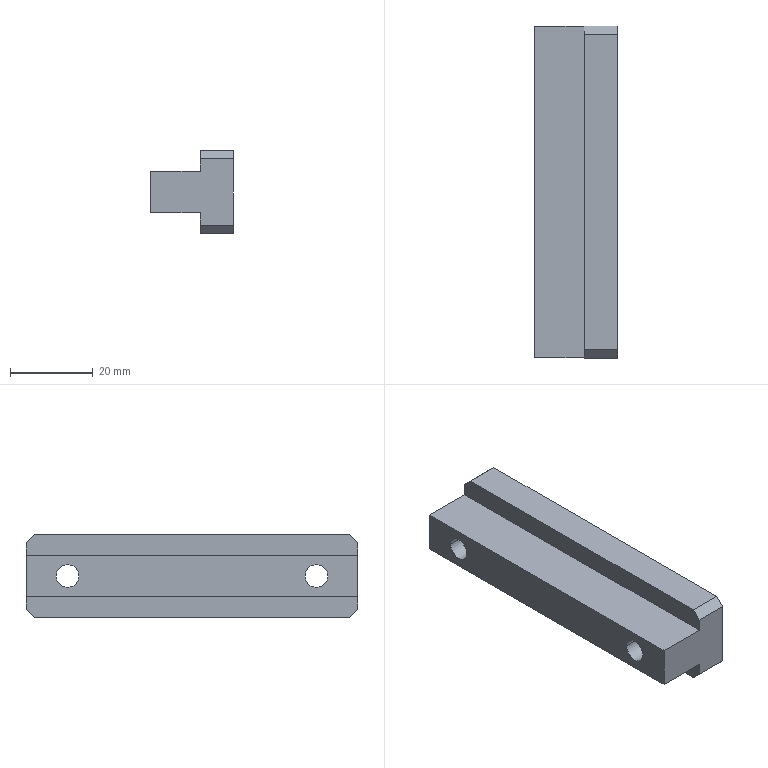Component | SolidWorks | ClampingAssembly-1_A85-1 | 1 solid | 24 faces | box 20 x 80 x 20 mm | volume 20761 mm3 | plane 16 | cylinder 8 | commonest cylinder face diameters 10 x4 5.5 x4 | material S136
build123d program:
from build123d import *

# Parameters (mm, degrees)
SKETCH1_W                                           = 80
SKETCH1_H                                           = 15
BOSS_EXTRUDE1_DEPTH                                 = 10
SKETCH2_W                                           = 12
SKETCH2_H                                           = 5
CUT_EXTRUDE1_DEPTH                                  = 81.971
SKETCH5_W                                           = 8
SKETCH5_H                                           = 5
BOSS_EXTRUDE2_DEPTH                                 = 80
HOLE_SIZE_ACCORDING_TO_HEXAGON_SOCKET_H_D           = 5.5
HOLE_SIZE_ACCORDING_TO_HEXAGON_SOCKET_H_CBORE_D     = 10
HOLE_SIZE_ACCORDING_TO_HEXAGON_SOCKET_H_CBORE_DEPTH = 5.7
CHAMFER1_SIZE                                       = 2


with BuildPart() as part:
    # Sketch1 → Boss-Extrude1 (new, symmetric)
    with BuildSketch(Plane(origin=(0, 0, 0), x_dir=(0, 0, -1), z_dir=(1, 0, 0))):
        Rectangle(SKETCH1_W, SKETCH1_H)
    extrude(amount=BOSS_EXTRUDE1_DEPTH, both=True)

    # Sketch2 → Cut-Extrude1 (cut, through all)
    with BuildSketch(Plane(origin=(0, 0, -40), x_dir=(-1, 0, 0), z_dir=(0, 0, -1))):
        with Locations((4, -5)):
            Rectangle(SKETCH2_W, SKETCH2_H)
    extrude(amount=-CUT_EXTRUDE1_DEPTH, mode=Mode.SUBTRACT)

    # Sketch5 → Boss-Extrude2 (add)
    with BuildSketch(Plane.XY.offset(40)):
        with Locations((6, 10)):
            Rectangle(SKETCH5_W, SKETCH5_H)
    extrude(amount=-BOSS_EXTRUDE2_DEPTH)

    # Hole Size_ according to_Hexagon Socket H (through all)
    with Locations(Plane(origin=(10, 0, 0), x_dir=(0, 0, -1), z_dir=(1, 0, 0))):
        with Locations((-30, 2.5), (30, 2.5)):
            CounterBoreHole(HOLE_SIZE_ACCORDING_TO_HEXAGON_SOCKET_H_D / 2, HOLE_SIZE_ACCORDING_TO_HEXAGON_SOCKET_H_CBORE_D / 2, HOLE_SIZE_ACCORDING_TO_HEXAGON_SOCKET_H_CBORE_DEPTH)

    # Chamfer1
    chamfer1_edges = [part.edges().sort_by_distance(p)[0] for p in [
        (6, 12.5, 40),
        (6, 12.5, -40),
        (6, -7.5, -40),
        (6, -7.5, 40),
    ]]
    chamfer(chamfer1_edges, length=CHAMFER1_SIZE)


solid = part.part

# Placed as in the assembly
solid = solid.moved(Location((-4.551, 48.036, -3), (90, 0, 0)))
STEP:
#1=CARTESIAN_POINT('',(-0.009873,0.5132,-0.01969));
#2=VERTEX_POINT('',#1);
#3=CARTESIAN_POINT('',(-0.009873,0.9069,-0.01969));
#4=VERTEX_POINT('',#3);
#5=CARTESIAN_POINT('',(-0.009873,0.7101,-0.01969));
#6=DIRECTION('',(1.,0.,-0.));
#7=DIRECTION('',(-0.,1.,0.));
#8=AXIS2_PLACEMENT_3D('',#5,#6,#7);
#9=CIRCLE('',#8,0.1969);
#10=EDGE_CURVE('',#2,#4,#9,.T.);
#11=ORIENTED_EDGE('',*,*,#10,.F.);
#12=CARTESIAN_POINT('',(0.2145,0.5132,-0.01969));
#13=VERTEX_POINT('',#12);
#14=CARTESIAN_POINT('',(0.2145,0.5132,-0.01969));
#15=DIRECTION('',(1.,0.,-0.));
#16=VECTOR('',#15,39.37);
#17=LINE('',#14,#16);
#18=EDGE_CURVE('',#2,#13,#17,.T.);
#19=ORIENTED_EDGE('',*,*,#18,.T.);
#20=CARTESIAN_POINT('',(0.2145,0.9069,-0.01969));
#21=VERTEX_POINT('',#20);
#22=CARTESIAN_POINT('',(0.2145,0.7101,-0.01969));
#23=DIRECTION('',(1.,0.,-0.));
#24=DIRECTION('',(-0.,1.,0.));
#25=AXIS2_PLACEMENT_3D('',#22,#23,#24);
#26=CIRCLE('',#25,0.1969);
#27=EDGE_CURVE('',#13,#21,#26,.T.);
#28=ORIENTED_EDGE('',*,*,#27,.T.);
#29=CARTESIAN_POINT('',(0.2145,0.9069,-0.01969));
#30=DIRECTION('',(1.,0.,-0.));
#31=VECTOR('',#30,39.37);
#32=LINE('',#29,#31);
#33=EDGE_CURVE('',#4,#21,#32,.T.);
#34=ORIENTED_EDGE('',*,*,#33,.F.);
#35=EDGE_LOOP('',(#11,#19,#28,#34));
#36=FACE_OUTER_BOUND('',#35,.T.);
#37=CARTESIAN_POINT('',(0.2145,0.7101,-0.01969));
#38=DIRECTION('',(1.,0.,-0.));
#39=DIRECTION('',(-0.,1.,0.));
#40=AXIS2_PLACEMENT_3D('',#37,#38,#39);
#41=CYLINDRICAL_SURFACE('',#40,0.1969);
#42=ADVANCED_FACE('',(#36),#41,.F.);
#43=CARTESIAN_POINT('',(-0.5729,0.6018,-0.01969));
#44=VERTEX_POINT('',#43);
#45=CARTESIAN_POINT('',(-0.5729,0.8183,-0.01969));
#46=VERTEX_POINT('',#45);
#47=CARTESIAN_POINT('',(-0.5729,0.7101,-0.01969));
#48=DIRECTION('',(1.,0.,-0.));
#49=DIRECTION('',(0.,1.,0.));
#50=AXIS2_PLACEMENT_3D('',#47,#48,#49);
#51=CIRCLE('',#50,0.1083);
#52=EDGE_CURVE('',#44,#46,#51,.T.);
#53=ORIENTED_EDGE('',*,*,#52,.F.);
#54=CARTESIAN_POINT('',(-0.009873,0.6018,-0.01969));
#55=VERTEX_POINT('',#54);
#56=CARTESIAN_POINT('',(0.2145,0.6018,-0.01969));
#57=DIRECTION('',(1.,0.,-0.));
#58=VECTOR('',#57,39.37);
#59=LINE('',#56,#58);
#60=EDGE_CURVE('',#44,#55,#59,.T.);
#61=ORIENTED_EDGE('',*,*,#60,.T.);
#62=CARTESIAN_POINT('',(-0.009873,0.8183,-0.01969));
#63=VERTEX_POINT('',#62);
#64=CARTESIAN_POINT('',(-0.009873,0.7101,-0.01969));
#65=DIRECTION('',(1.,0.,-0.));
#66=DIRECTION('',(-0.,1.,0.));
#67=AXIS2_PLACEMENT_3D('',#64,#65,#66);
#68=CIRCLE('',#67,0.1083);
#69=EDGE_CURVE('',#55,#63,#68,.T.);
#70=ORIENTED_EDGE('',*,*,#69,.T.);
#71=CARTESIAN_POINT('',(0.2145,0.8183,-0.01969));
#72=DIRECTION('',(1.,0.,-0.));
#73=VECTOR('',#72,39.37);
#74=LINE('',#71,#73);
#75=EDGE_CURVE('',#46,#63,#74,.T.);
#76=ORIENTED_EDGE('',*,*,#75,.F.);
#77=EDGE_LOOP('',(#53,#61,#70,#76));
#78=FACE_OUTER_BOUND('',#77,.T.);
#79=CARTESIAN_POINT('',(0.2145,0.7101,-0.01969));
#80=DIRECTION('',(1.,0.,-0.));
#81=DIRECTION('',(0.,1.,0.));
#82=AXIS2_PLACEMENT_3D('',#79,#80,#81);
#83=CYLINDRICAL_SURFACE('',#82,0.1083);
#84=ADVANCED_FACE('',(#78),#83,.F.);
#85=CARTESIAN_POINT('',(-0.009873,2.875,-0.01969));
#86=VERTEX_POINT('',#85);
#87=CARTESIAN_POINT('',(-0.009873,3.269,-0.01969));
#88=VERTEX_POINT('',#87);
#89=CARTESIAN_POINT('',(-0.009873,3.072,-0.01969));
#90=DIRECTION('',(1.,0.,-0.));
#91=DIRECTION('',(-0.,1.,0.));
#92=AXIS2_PLACEMENT_3D('',#89,#90,#91);
#93=CIRCLE('',#92,0.1969);
#94=EDGE_CURVE('',#86,#88,#93,.T.);
#95=ORIENTED_EDGE('',*,*,#94,.F.);
#96=CARTESIAN_POINT('',(0.2145,2.875,-0.01969));
#97=VERTEX_POINT('',#96);
#98=CARTESIAN_POINT('',(0.2145,2.875,-0.01969));
#99=DIRECTION('',(1.,0.,-0.));
#100=VECTOR('',#99,39.37);
#101=LINE('',#98,#100);
#102=EDGE_CURVE('',#86,#97,#101,.T.);
#103=ORIENTED_EDGE('',*,*,#102,.T.);
#104=CARTESIAN_POINT('',(0.2145,3.269,-0.01969));
#105=VERTEX_POINT('',#104);
#106=CARTESIAN_POINT('',(0.2145,3.072,-0.01969));
#107=DIRECTION('',(1.,0.,-0.));
#108=DIRECTION('',(-0.,1.,0.));
#109=AXIS2_PLACEMENT_3D('',#106,#107,#108);
#110=CIRCLE('',#109,0.1969);
#111=EDGE_CURVE('',#97,#105,#110,.T.);
#112=ORIENTED_EDGE('',*,*,#111,.T.);
#113=CARTESIAN_POINT('',(0.2145,3.269,-0.01969));
#114=DIRECTION('',(1.,0.,-0.));
#115=VECTOR('',#114,39.37);
#116=LINE('',#113,#115);
#117=EDGE_CURVE('',#88,#105,#116,.T.);
#118=ORIENTED_EDGE('',*,*,#117,.F.);
#119=EDGE_LOOP('',(#95,#103,#112,#118));
#120=FACE_OUTER_BOUND('',#119,.T.);
#121=CARTESIAN_POINT('',(0.2145,3.072,-0.01969));
#122=DIRECTION('',(1.,0.,-0.));
#123=DIRECTION('',(-0.,1.,0.));
#124=AXIS2_PLACEMENT_3D('',#121,#122,#123);
#125=CYLINDRICAL_SURFACE('',#124,0.1969);
#126=ADVANCED_FACE('',(#120),#125,.F.);
#127=CARTESIAN_POINT('',(-0.5729,2.964,-0.01969));
#128=VERTEX_POINT('',#127);
#129=CARTESIAN_POINT('',(-0.5729,3.181,-0.01969));
#130=VERTEX_POINT('',#129);
#131=CARTESIAN_POINT('',(-0.5729,3.072,-0.01969));
#132=DIRECTION('',(1.,0.,-0.));
#133=DIRECTION('',(0.,1.,0.));
#134=AXIS2_PLACEMENT_3D('',#131,#132,#133);
#135=CIRCLE('',#134,0.1083);
#136=EDGE_CURVE('',#128,#130,#135,.T.);
#137=ORIENTED_EDGE('',*,*,#136,.F.);
#138=CARTESIAN_POINT('',(-0.009873,2.964,-0.01969));
#139=VERTEX_POINT('',#138);
#140=CARTESIAN_POINT('',(0.2145,2.964,-0.01969));
#141=DIRECTION('',(1.,0.,-0.));
#142=VECTOR('',#141,39.37);
#143=LINE('',#140,#142);
#144=EDGE_CURVE('',#128,#139,#143,.T.);
#145=ORIENTED_EDGE('',*,*,#144,.T.);
#146=CARTESIAN_POINT('',(-0.009873,3.181,-0.01969));
#147=VERTEX_POINT('',#146);
#148=CARTESIAN_POINT('',(-0.009873,3.072,-0.01969));
#149=DIRECTION('',(1.,0.,-0.));
#150=DIRECTION('',(-0.,1.,0.));
#151=AXIS2_PLACEMENT_3D('',#148,#149,#150);
#152=CIRCLE('',#151,0.1083);
#153=EDGE_CURVE('',#139,#147,#152,.T.);
#154=ORIENTED_EDGE('',*,*,#153,.T.);
#155=CARTESIAN_POINT('',(0.2145,3.181,-0.01969));
#156=DIRECTION('',(1.,0.,-0.));
#157=VECTOR('',#156,39.37);
#158=LINE('',#155,#157);
#159=EDGE_CURVE('',#130,#147,#158,.T.);
#160=ORIENTED_EDGE('',*,*,#159,.F.);
#161=EDGE_LOOP('',(#137,#145,#154,#160));
#162=FACE_OUTER_BOUND('',#161,.T.);
#163=CARTESIAN_POINT('',(0.2145,3.072,-0.01969));
#164=DIRECTION('',(1.,0.,-0.));
#165=DIRECTION('',(0.,1.,0.));
#166=AXIS2_PLACEMENT_3D('',#163,#164,#165);
#167=CYLINDRICAL_SURFACE('',#166,0.1083);
#168=ADVANCED_FACE('',(#162),#167,.F.);
#169=CARTESIAN_POINT('',(-0.1004,3.466,0.1772));
#170=VERTEX_POINT('',#169);
#171=CARTESIAN_POINT('',(-0.1004,0.3164,0.1772));
#172=VERTEX_POINT('',#171);
#173=CARTESIAN_POINT('',(-0.1004,3.837,0.1772));
#174=DIRECTION('',(0.,-1.,-0.));
#175=VECTOR('',#174,39.37);
#176=LINE('',#173,#175);
#177=EDGE_CURVE('',#170,#172,#176,.T.);
#178=ORIENTED_EDGE('',*,*,#177,.F.);
#179=CARTESIAN_POINT('',(-0.5729,3.466,0.1772));
#180=VERTEX_POINT('',#179);
#181=CARTESIAN_POINT('',(0.2145,3.466,0.1772));
#182=DIRECTION('',(-1.,-0.,0.));
#183=VECTOR('',#182,39.37);
#184=LINE('',#181,#183);
#185=EDGE_CURVE('',#170,#180,#184,.T.);
#186=ORIENTED_EDGE('',*,*,#185,.T.);
#187=CARTESIAN_POINT('',(-0.5729,0.3164,0.1772));
#188=VERTEX_POINT('',#187);
#189=CARTESIAN_POINT('',(-0.5729,0.3164,0.1772));
#190=DIRECTION('',(0.,-1.,-0.));
#191=VECTOR('',#190,39.37);
#192=LINE('',#189,#191);
#193=EDGE_CURVE('',#180,#188,#192,.T.);
#194=ORIENTED_EDGE('',*,*,#193,.T.);
#195=CARTESIAN_POINT('',(0.2145,0.3164,0.1772));
#196=DIRECTION('',(-1.,-0.,0.));
#197=VECTOR('',#196,39.37);
#198=LINE('',#195,#197);
#199=EDGE_CURVE('',#172,#188,#198,.T.);
#200=ORIENTED_EDGE('',*,*,#199,.F.);
#201=EDGE_LOOP('',(#178,#186,#194,#200));
#202=FACE_OUTER_BOUND('',#201,.T.);
#203=CARTESIAN_POINT('',(0.2145,0.3164,0.1772));
#204=DIRECTION('',(-0.,0.,-1.));
#205=DIRECTION('',(-0.,1.,0.));
#206=AXIS2_PLACEMENT_3D('',#203,#204,#205);
#207=PLANE('',#206);
#208=ADVANCED_FACE('',(#202),#207,.F.);
#209=CARTESIAN_POINT('',(0.2145,3.466,-0.3346));
#210=VERTEX_POINT('',#209);
#211=CARTESIAN_POINT('',(0.2145,3.466,0.2953));
#212=VERTEX_POINT('',#211);
#213=CARTESIAN_POINT('',(0.2145,3.466,0.1772));
#214=DIRECTION('',(0.,-0.,1.));
#215=VECTOR('',#214,39.37);
#216=LINE('',#213,#215);
#217=EDGE_CURVE('',#210,#212,#216,.T.);
#218=ORIENTED_EDGE('',*,*,#217,.F.);
#219=CARTESIAN_POINT('',(-0.1004,3.466,-0.3346));
#220=VERTEX_POINT('',#219);
#221=CARTESIAN_POINT('',(0.2145,3.466,-0.3346));
#222=DIRECTION('',(-1.,-0.,0.));
#223=VECTOR('',#222,39.37);
#224=LINE('',#221,#223);
#225=EDGE_CURVE('',#210,#220,#224,.T.);
#226=ORIENTED_EDGE('',*,*,#225,.T.);
#227=CARTESIAN_POINT('',(-0.1004,3.466,-0.2165));
#228=VERTEX_POINT('',#227);
#229=CARTESIAN_POINT('',(-0.1004,3.466,-0.4134));
#230=DIRECTION('',(-0.,0.,-1.));
#231=VECTOR('',#230,39.37);
#232=LINE('',#229,#231);
#233=EDGE_CURVE('',#228,#220,#232,.T.);
#234=ORIENTED_EDGE('',*,*,#233,.F.);
#235=CARTESIAN_POINT('',(-0.5729,3.466,-0.2165));
#236=VERTEX_POINT('',#235);
#237=CARTESIAN_POINT('',(-0.5729,3.466,-0.2165));
#238=DIRECTION('',(1.,0.,-0.));
#239=VECTOR('',#238,39.37);
#240=LINE('',#237,#239);
#241=EDGE_CURVE('',#236,#228,#240,.T.);
#242=ORIENTED_EDGE('',*,*,#241,.F.);
#243=CARTESIAN_POINT('',(-0.5729,3.466,0.1772));
#244=DIRECTION('',(0.,-0.,1.));
#245=VECTOR('',#244,39.37);
#246=LINE('',#243,#245);
#247=EDGE_CURVE('',#236,#180,#246,.T.);
#248=ORIENTED_EDGE('',*,*,#247,.T.);
#249=ORIENTED_EDGE('',*,*,#185,.F.);
#250=CARTESIAN_POINT('',(-0.1004,3.466,0.2953));
#251=VERTEX_POINT('',#250);
#252=CARTESIAN_POINT('',(-0.1004,3.466,0.1772));
#253=DIRECTION('',(0.,-0.,1.));
#254=VECTOR('',#253,39.37);
#255=LINE('',#252,#254);
#256=EDGE_CURVE('',#170,#251,#255,.T.);
#257=ORIENTED_EDGE('',*,*,#256,.T.);
#258=CARTESIAN_POINT('',(0.2145,3.466,0.2953));
#259=DIRECTION('',(1.,0.,-0.));
#260=VECTOR('',#259,39.37);
#261=LINE('',#258,#260);
#262=EDGE_CURVE('',#251,#212,#261,.T.);
#263=ORIENTED_EDGE('',*,*,#262,.T.);
#264=EDGE_LOOP('',(#218,#226,#234,#242,#248,#249,#257,#263));
#265=FACE_OUTER_BOUND('',#264,.T.);
#266=CARTESIAN_POINT('',(0.2145,3.466,0.1772));
#267=DIRECTION('',(0.,-1.,-0.));
#268=DIRECTION('',(-0.,0.,-1.));
#269=AXIS2_PLACEMENT_3D('',#266,#267,#268);
#270=PLANE('',#269);
#271=ADVANCED_FACE('',(#265),#270,.F.);
#272=CARTESIAN_POINT('',(0.2145,0.3164,0.2953));
#273=VERTEX_POINT('',#272);
#274=CARTESIAN_POINT('',(0.2145,0.3164,-0.3346));
#275=VERTEX_POINT('',#274);
#276=CARTESIAN_POINT('',(0.2145,0.3164,0.1772));
#277=DIRECTION('',(-0.,-0.,-1.));
#278=VECTOR('',#277,39.37);
#279=LINE('',#276,#278);
#280=EDGE_CURVE('',#273,#275,#279,.T.);
#281=ORIENTED_EDGE('',*,*,#280,.F.);
#282=CARTESIAN_POINT('',(-0.1004,0.3164,0.2953));
#283=VERTEX_POINT('',#282);
#284=CARTESIAN_POINT('',(-0.1004,0.3164,0.2953));
#285=DIRECTION('',(-1.,-0.,0.));
#286=VECTOR('',#285,39.37);
#287=LINE('',#284,#286);
#288=EDGE_CURVE('',#273,#283,#287,.T.);
#289=ORIENTED_EDGE('',*,*,#288,.T.);
#290=CARTESIAN_POINT('',(-0.1004,0.3164,0.1772));
#291=DIRECTION('',(-0.,0.,-1.));
#292=VECTOR('',#291,39.37);
#293=LINE('',#290,#292);
#294=EDGE_CURVE('',#283,#172,#293,.T.);
#295=ORIENTED_EDGE('',*,*,#294,.T.);
#296=ORIENTED_EDGE('',*,*,#199,.T.);
#297=CARTESIAN_POINT('',(-0.5729,0.3164,-0.2165));
#298=VERTEX_POINT('',#297);
#299=CARTESIAN_POINT('',(-0.5729,0.3164,0.1772));
#300=DIRECTION('',(-0.,-0.,-1.));
#301=VECTOR('',#300,39.37);
#302=LINE('',#299,#301);
#303=EDGE_CURVE('',#188,#298,#302,.T.);
#304=ORIENTED_EDGE('',*,*,#303,.T.);
#305=CARTESIAN_POINT('',(-0.1004,0.3164,-0.2165));
#306=VERTEX_POINT('',#305);
#307=CARTESIAN_POINT('',(-0.5729,0.3164,-0.2165));
#308=DIRECTION('',(1.,0.,-0.));
#309=VECTOR('',#308,39.37);
#310=LINE('',#307,#309);
#311=EDGE_CURVE('',#298,#306,#310,.T.);
#312=ORIENTED_EDGE('',*,*,#311,.T.);
#313=CARTESIAN_POINT('',(-0.1004,0.3164,-0.3346));
#314=VERTEX_POINT('',#313);
#315=CARTESIAN_POINT('',(-0.1004,0.3164,-0.4134));
#316=DIRECTION('',(-0.,0.,-1.));
#317=VECTOR('',#316,39.37);
#318=LINE('',#315,#317);
#319=EDGE_CURVE('',#306,#314,#318,.T.);
#320=ORIENTED_EDGE('',*,*,#319,.T.);
#321=CARTESIAN_POINT('',(0.2145,0.3164,-0.3346));
#322=DIRECTION('',(1.,0.,-0.));
#323=VECTOR('',#322,39.37);
#324=LINE('',#321,#323);
#325=EDGE_CURVE('',#314,#275,#324,.T.);
#326=ORIENTED_EDGE('',*,*,#325,.T.);
#327=EDGE_LOOP('',(#281,#289,#295,#296,#304,#312,#320,#326));
#328=FACE_OUTER_BOUND('',#327,.T.);
#329=CARTESIAN_POINT('',(0.2145,0.3164,0.1772));
#330=DIRECTION('',(-0.,1.,-0.));
#331=DIRECTION('',(0.,0.,1.));
#332=AXIS2_PLACEMENT_3D('',#329,#330,#331);
#333=PLANE('',#332);
#334=ADVANCED_FACE('',(#328),#333,.F.);
#335=CARTESIAN_POINT('',(-0.1004,0.3951,-0.4134));
#336=VERTEX_POINT('',#335);
#337=CARTESIAN_POINT('',(-0.1004,3.387,-0.4134));
#338=VERTEX_POINT('',#337);
#339=CARTESIAN_POINT('',(-0.1004,0.3164,-0.4134));
#340=DIRECTION('',(-0.,1.,0.));
#341=VECTOR('',#340,39.37);
#342=LINE('',#339,#341);
#343=EDGE_CURVE('',#336,#338,#342,.T.);
#344=ORIENTED_EDGE('',*,*,#343,.T.);
#345=CARTESIAN_POINT('',(0.2145,3.387,-0.4134));
#346=VERTEX_POINT('',#345);
#347=CARTESIAN_POINT('',(0.2145,3.387,-0.4134));
#348=DIRECTION('',(1.,0.,-0.));
#349=VECTOR('',#348,39.37);
#350=LINE('',#347,#349);
#351=EDGE_CURVE('',#338,#346,#350,.T.);
#352=ORIENTED_EDGE('',*,*,#351,.T.);
#353=CARTESIAN_POINT('',(0.2145,0.3951,-0.4134));
#354=VERTEX_POINT('',#353);
#355=CARTESIAN_POINT('',(0.2145,0.3164,-0.4134));
#356=DIRECTION('',(-0.,1.,0.));
#357=VECTOR('',#356,39.37);
#358=LINE('',#355,#357);
#359=EDGE_CURVE('',#354,#346,#358,.T.);
#360=ORIENTED_EDGE('',*,*,#359,.F.);
#361=CARTESIAN_POINT('',(0.2145,0.3951,-0.4134));
#362=DIRECTION('',(-1.,-0.,0.));
#363=VECTOR('',#362,39.37);
#364=LINE('',#361,#363);
#365=EDGE_CURVE('',#354,#336,#364,.T.);
#366=ORIENTED_EDGE('',*,*,#365,.T.);
#367=EDGE_LOOP('',(#344,#352,#360,#366));
#368=FACE_OUTER_BOUND('',#367,.T.);
#369=CARTESIAN_POINT('',(0.2145,0.3164,-0.4134));
#370=DIRECTION('',(0.,-0.,1.));
#371=DIRECTION('',(0.,-1.,-0.));
#372=AXIS2_PLACEMENT_3D('',#369,#370,#371);
#373=PLANE('',#372);
#374=ADVANCED_FACE('',(#368),#373,.F.);
#375=CARTESIAN_POINT('',(0.2145,0.7101,-0.01969));
#376=DIRECTION('',(1.,0.,-0.));
#377=DIRECTION('',(-0.,1.,0.));
#378=AXIS2_PLACEMENT_3D('',#375,#376,#377);
#379=CIRCLE('',#378,0.1969);
#380=EDGE_CURVE('',#21,#13,#379,.T.);
#381=ORIENTED_EDGE('',*,*,#380,.F.);
#382=ORIENTED_EDGE('',*,*,#27,.F.);
#383=EDGE_LOOP('',(#381,#382));
#384=FACE_BOUND('',#383,.T.);
#385=CARTESIAN_POINT('',(0.2145,3.072,-0.01969));
#386=DIRECTION('',(1.,0.,-0.));
#387=DIRECTION('',(-0.,1.,0.));
#388=AXIS2_PLACEMENT_3D('',#385,#386,#387);
#389=CIRCLE('',#388,0.1969);
#390=EDGE_CURVE('',#105,#97,#389,.T.);
#391=ORIENTED_EDGE('',*,*,#390,.F.);
#392=ORIENTED_EDGE('',*,*,#111,.F.);
#393=EDGE_LOOP('',(#391,#392));
#394=FACE_BOUND('',#393,.T.);
#395=ORIENTED_EDGE('',*,*,#359,.T.);
#396=CARTESIAN_POINT('',(0.2145,2.787,-1.014));
#397=DIRECTION('',(0.,0.7071,0.7071));
#398=VECTOR('',#397,39.37);
#399=LINE('',#396,#398);
#400=EDGE_CURVE('',#346,#210,#399,.T.);
#401=ORIENTED_EDGE('',*,*,#400,.T.);
#402=ORIENTED_EDGE('',*,*,#217,.T.);
#403=CARTESIAN_POINT('',(0.2145,3.387,0.374));
#404=VERTEX_POINT('',#403);
#405=CARTESIAN_POINT('',(0.2145,2.885,0.876));
#406=DIRECTION('',(0.,-0.7071,0.7071));
#407=VECTOR('',#406,39.37);
#408=LINE('',#405,#407);
#409=EDGE_CURVE('',#212,#404,#408,.T.);
#410=ORIENTED_EDGE('',*,*,#409,.T.);
#411=CARTESIAN_POINT('',(0.2145,0.3951,0.374));
#412=VERTEX_POINT('',#411);
#413=CARTESIAN_POINT('',(0.2145,3.837,0.374));
#414=DIRECTION('',(0.,-1.,-0.));
#415=VECTOR('',#414,39.37);
#416=LINE('',#413,#415);
#417=EDGE_CURVE('',#404,#412,#416,.T.);
#418=ORIENTED_EDGE('',*,*,#417,.T.);
#419=CARTESIAN_POINT('',(0.2145,0.8971,0.876));
#420=DIRECTION('',(-0.,-0.7071,-0.7071));
#421=VECTOR('',#420,39.37);
#422=LINE('',#419,#421);
#423=EDGE_CURVE('',#412,#273,#422,.T.);
#424=ORIENTED_EDGE('',*,*,#423,.T.);
#425=ORIENTED_EDGE('',*,*,#280,.T.);
#426=CARTESIAN_POINT('',(0.2145,0.9955,-1.014));
#427=DIRECTION('',(-0.,0.7071,-0.7071));
#428=VECTOR('',#427,39.37);
#429=LINE('',#426,#428);
#430=EDGE_CURVE('',#275,#354,#429,.T.);
#431=ORIENTED_EDGE('',*,*,#430,.T.);
#432=EDGE_LOOP('',(#395,#401,#402,#410,#418,#424,#425,#431));
#433=FACE_OUTER_BOUND('',#432,.T.);
#434=CARTESIAN_POINT('',(0.2145,1.891,-0.1181));
#435=DIRECTION('',(1.,0.,-0.));
#436=DIRECTION('',(-0.,1.,0.));
#437=AXIS2_PLACEMENT_3D('',#434,#435,#436);
#438=PLANE('',#437);
#439=ADVANCED_FACE('',(#384,#394,#433),#438,.T.);
#440=CARTESIAN_POINT('',(-0.5729,0.7101,-0.01969));
#441=DIRECTION('',(1.,0.,-0.));
#442=DIRECTION('',(0.,1.,0.));
#443=AXIS2_PLACEMENT_3D('',#440,#441,#442);
#444=CIRCLE('',#443,0.1083);
#445=EDGE_CURVE('',#46,#44,#444,.T.);
#446=ORIENTED_EDGE('',*,*,#445,.T.);
#447=ORIENTED_EDGE('',*,*,#52,.T.);
#448=EDGE_LOOP('',(#446,#447));
#449=FACE_BOUND('',#448,.T.);
#450=CARTESIAN_POINT('',(-0.5729,3.072,-0.01969));
#451=DIRECTION('',(1.,0.,-0.));
#452=DIRECTION('',(0.,1.,0.));
#453=AXIS2_PLACEMENT_3D('',#450,#451,#452);
#454=CIRCLE('',#453,0.1083);
#455=EDGE_CURVE('',#130,#128,#454,.T.);
#456=ORIENTED_EDGE('',*,*,#455,.T.);
#457=ORIENTED_EDGE('',*,*,#136,.T.);
#458=EDGE_LOOP('',(#456,#457));
#459=FACE_BOUND('',#458,.T.);
#460=ORIENTED_EDGE('',*,*,#247,.F.);
#461=CARTESIAN_POINT('',(-0.5729,0.3164,-0.2165));
#462=DIRECTION('',(-0.,1.,0.));
#463=VECTOR('',#462,39.37);
#464=LINE('',#461,#463);
#465=EDGE_CURVE('',#298,#236,#464,.T.);
#466=ORIENTED_EDGE('',*,*,#465,.F.);
#467=ORIENTED_EDGE('',*,*,#303,.F.);
#468=ORIENTED_EDGE('',*,*,#193,.F.);
#469=EDGE_LOOP('',(#460,#466,#467,#468));
#470=FACE_OUTER_BOUND('',#469,.T.);
#471=CARTESIAN_POINT('',(-0.5729,1.891,-0.1181));
#472=DIRECTION('',(1.,0.,-0.));
#473=DIRECTION('',(-0.,1.,0.));
#474=AXIS2_PLACEMENT_3D('',#471,#472,#473);
#475=PLANE('',#474);
#476=ADVANCED_FACE('',(#449,#459,#470),#475,.F.);
#477=ORIENTED_EDGE('',*,*,#233,.T.);
#478=CARTESIAN_POINT('',(-0.1004,3.466,-0.3346));
#479=DIRECTION('',(-0.,-0.7071,-0.7071));
#480=VECTOR('',#479,39.37);
#481=LINE('',#478,#480);
#482=EDGE_CURVE('',#220,#338,#481,.T.);
#483=ORIENTED_EDGE('',*,*,#482,.T.);
#484=ORIENTED_EDGE('',*,*,#343,.F.);
#485=CARTESIAN_POINT('',(-0.1004,0.3951,-0.4134));
#486=DIRECTION('',(0.,-0.7071,0.7071));
#487=VECTOR('',#486,39.37);
#488=LINE('',#485,#487);
#489=EDGE_CURVE('',#336,#314,#488,.T.);
#490=ORIENTED_EDGE('',*,*,#489,.T.);
#491=ORIENTED_EDGE('',*,*,#319,.F.);
#492=CARTESIAN_POINT('',(-0.1004,0.3164,-0.2165));
#493=DIRECTION('',(-0.,1.,0.));
#494=VECTOR('',#493,39.37);
#495=LINE('',#492,#494);
#496=EDGE_CURVE('',#306,#228,#495,.T.);
#497=ORIENTED_EDGE('',*,*,#496,.T.);
#498=EDGE_LOOP('',(#477,#483,#484,#490,#491,#497));
#499=FACE_OUTER_BOUND('',#498,.T.);
#500=CARTESIAN_POINT('',(-0.1004,0.3164,-0.4134));
#501=DIRECTION('',(1.,0.,-0.));
#502=DIRECTION('',(-0.,1.,0.));
#503=AXIS2_PLACEMENT_3D('',#500,#501,#502);
#504=PLANE('',#503);
#505=ADVANCED_FACE('',(#499),#504,.F.);
#506=ORIENTED_EDGE('',*,*,#241,.T.);
#507=ORIENTED_EDGE('',*,*,#496,.F.);
#508=ORIENTED_EDGE('',*,*,#311,.F.);
#509=ORIENTED_EDGE('',*,*,#465,.T.);
#510=EDGE_LOOP('',(#506,#507,#508,#509));
#511=FACE_OUTER_BOUND('',#510,.T.);
#512=CARTESIAN_POINT('',(-0.5729,0.3164,-0.2165));
#513=DIRECTION('',(0.,-0.,1.));
#514=DIRECTION('',(0.,-1.,-0.));
#515=AXIS2_PLACEMENT_3D('',#512,#513,#514);
#516=PLANE('',#515);
#517=ADVANCED_FACE('',(#511),#516,.F.);
#518=CARTESIAN_POINT('',(-0.1004,3.387,0.374));
#519=VERTEX_POINT('',#518);
#520=CARTESIAN_POINT('',(-0.1004,0.3951,0.374));
#521=VERTEX_POINT('',#520);
#522=CARTESIAN_POINT('',(-0.1004,3.837,0.374));
#523=DIRECTION('',(0.,-1.,-0.));
#524=VECTOR('',#523,39.37);
#525=LINE('',#522,#524);
#526=EDGE_CURVE('',#519,#521,#525,.T.);
#527=ORIENTED_EDGE('',*,*,#526,.F.);
#528=CARTESIAN_POINT('',(-0.1004,3.711,0.05051));
#529=DIRECTION('',(-0.,0.7071,-0.7071));
#530=VECTOR('',#529,39.37);
#531=LINE('',#528,#530);
#532=EDGE_CURVE('',#519,#251,#531,.T.);
#533=ORIENTED_EDGE('',*,*,#532,.T.);
#534=ORIENTED_EDGE('',*,*,#256,.F.);
#535=ORIENTED_EDGE('',*,*,#177,.T.);
#536=ORIENTED_EDGE('',*,*,#294,.F.);
#537=CARTESIAN_POINT('',(-0.1004,2.018,1.997));
#538=DIRECTION('',(0.,0.7071,0.7071));
#539=VECTOR('',#538,39.37);
#540=LINE('',#537,#539);
#541=EDGE_CURVE('',#283,#521,#540,.T.);
#542=ORIENTED_EDGE('',*,*,#541,.T.);
#543=EDGE_LOOP('',(#527,#533,#534,#535,#536,#542));
#544=FACE_OUTER_BOUND('',#543,.T.);
#545=CARTESIAN_POINT('',(-0.1004,3.837,0.1772));
#546=DIRECTION('',(-1.,-0.,0.));
#547=DIRECTION('',(0.,-1.,-0.));
#548=AXIS2_PLACEMENT_3D('',#545,#546,#547);
#549=PLANE('',#548);
#550=ADVANCED_FACE('',(#544),#549,.T.);
#551=ORIENTED_EDGE('',*,*,#417,.F.);
#552=CARTESIAN_POINT('',(-0.1004,3.387,0.374));
#553=DIRECTION('',(-1.,-0.,0.));
#554=VECTOR('',#553,39.37);
#555=LINE('',#552,#554);
#556=EDGE_CURVE('',#404,#519,#555,.T.);
#557=ORIENTED_EDGE('',*,*,#556,.T.);
#558=ORIENTED_EDGE('',*,*,#526,.T.);
#559=CARTESIAN_POINT('',(0.2145,0.3951,0.374));
#560=DIRECTION('',(1.,0.,-0.));
#561=VECTOR('',#560,39.37);
#562=LINE('',#559,#561);
#563=EDGE_CURVE('',#521,#412,#562,.T.);
#564=ORIENTED_EDGE('',*,*,#563,.T.);
#565=EDGE_LOOP('',(#551,#557,#558,#564));
#566=FACE_OUTER_BOUND('',#565,.T.);
#567=CARTESIAN_POINT('',(0.2145,3.837,0.374));
#568=DIRECTION('',(0.,-0.,1.));
#569=DIRECTION('',(0.,-1.,-0.));
#570=AXIS2_PLACEMENT_3D('',#567,#568,#569);
#571=PLANE('',#570);
#572=ADVANCED_FACE('',(#566),#571,.T.);
#573=ORIENTED_EDGE('',*,*,#144,.F.);
#574=ORIENTED_EDGE('',*,*,#455,.F.);
#575=ORIENTED_EDGE('',*,*,#159,.T.);
#576=CARTESIAN_POINT('',(-0.009873,3.072,-0.01969));
#577=DIRECTION('',(1.,0.,-0.));
#578=DIRECTION('',(-0.,1.,0.));
#579=AXIS2_PLACEMENT_3D('',#576,#577,#578);
#580=CIRCLE('',#579,0.1083);
#581=EDGE_CURVE('',#147,#139,#580,.T.);
#582=ORIENTED_EDGE('',*,*,#581,.T.);
#583=EDGE_LOOP('',(#573,#574,#575,#582));
#584=FACE_OUTER_BOUND('',#583,.T.);
#585=CARTESIAN_POINT('',(0.2145,3.072,-0.01969));
#586=DIRECTION('',(1.,0.,-0.));
#587=DIRECTION('',(0.,1.,0.));
#588=AXIS2_PLACEMENT_3D('',#585,#586,#587);
#589=CYLINDRICAL_SURFACE('',#588,0.1083);
#590=ADVANCED_FACE('',(#584),#589,.F.);
#591=ORIENTED_EDGE('',*,*,#581,.F.);
#592=ORIENTED_EDGE('',*,*,#153,.F.);
#593=EDGE_LOOP('',(#591,#592));
#594=FACE_BOUND('',#593,.T.);
#595=CARTESIAN_POINT('',(-0.009873,3.072,-0.01969));
#596=DIRECTION('',(1.,0.,-0.));
#597=DIRECTION('',(-0.,1.,0.));
#598=AXIS2_PLACEMENT_3D('',#595,#596,#597);
#599=CIRCLE('',#598,0.1969);
#600=EDGE_CURVE('',#88,#86,#599,.T.);
#601=ORIENTED_EDGE('',*,*,#600,.T.);
#602=ORIENTED_EDGE('',*,*,#94,.T.);
#603=EDGE_LOOP('',(#601,#602));
#604=FACE_OUTER_BOUND('',#603,.T.);
#605=CARTESIAN_POINT('',(-0.009873,3.072,0.08858));
#606=DIRECTION('',(-1.,-0.,0.));
#607=DIRECTION('',(0.,-1.,-0.));
#608=AXIS2_PLACEMENT_3D('',#605,#606,#607);
#609=PLANE('',#608);
#610=ADVANCED_FACE('',(#594,#604),#609,.F.);
#611=ORIENTED_EDGE('',*,*,#102,.F.);
#612=ORIENTED_EDGE('',*,*,#600,.F.);
#613=ORIENTED_EDGE('',*,*,#117,.T.);
#614=ORIENTED_EDGE('',*,*,#390,.T.);
#615=EDGE_LOOP('',(#611,#612,#613,#614));
#616=FACE_OUTER_BOUND('',#615,.T.);
#617=CARTESIAN_POINT('',(0.2145,3.072,-0.01969));
#618=DIRECTION('',(1.,0.,-0.));
#619=DIRECTION('',(-0.,1.,0.));
#620=AXIS2_PLACEMENT_3D('',#617,#618,#619);
#621=CYLINDRICAL_SURFACE('',#620,0.1969);
#622=ADVANCED_FACE('',(#616),#621,.F.);
#623=ORIENTED_EDGE('',*,*,#60,.F.);
#624=ORIENTED_EDGE('',*,*,#445,.F.);
#625=ORIENTED_EDGE('',*,*,#75,.T.);
#626=CARTESIAN_POINT('',(-0.009873,0.7101,-0.01969));
#627=DIRECTION('',(1.,0.,-0.));
#628=DIRECTION('',(-0.,1.,0.));
#629=AXIS2_PLACEMENT_3D('',#626,#627,#628);
#630=CIRCLE('',#629,0.1083);
#631=EDGE_CURVE('',#63,#55,#630,.T.);
#632=ORIENTED_EDGE('',*,*,#631,.T.);
#633=EDGE_LOOP('',(#623,#624,#625,#632));
#634=FACE_OUTER_BOUND('',#633,.T.);
#635=CARTESIAN_POINT('',(0.2145,0.7101,-0.01969));
#636=DIRECTION('',(1.,0.,-0.));
#637=DIRECTION('',(0.,1.,0.));
#638=AXIS2_PLACEMENT_3D('',#635,#636,#637);
#639=CYLINDRICAL_SURFACE('',#638,0.1083);
#640=ADVANCED_FACE('',(#634),#639,.F.);
#641=ORIENTED_EDGE('',*,*,#631,.F.);
#642=ORIENTED_EDGE('',*,*,#69,.F.);
#643=EDGE_LOOP('',(#641,#642));
#644=FACE_BOUND('',#643,.T.);
#645=CARTESIAN_POINT('',(-0.009873,0.7101,-0.01969));
#646=DIRECTION('',(1.,0.,-0.));
#647=DIRECTION('',(-0.,1.,0.));
#648=AXIS2_PLACEMENT_3D('',#645,#646,#647);
#649=CIRCLE('',#648,0.1969);
#650=EDGE_CURVE('',#4,#2,#649,.T.);
#651=ORIENTED_EDGE('',*,*,#650,.T.);
#652=ORIENTED_EDGE('',*,*,#10,.T.);
#653=EDGE_LOOP('',(#651,#652));
#654=FACE_OUTER_BOUND('',#653,.T.);
#655=CARTESIAN_POINT('',(-0.009873,0.7101,0.08858));
#656=DIRECTION('',(-1.,-0.,0.));
#657=DIRECTION('',(0.,-1.,-0.));
#658=AXIS2_PLACEMENT_3D('',#655,#656,#657);
#659=PLANE('',#658);
#660=ADVANCED_FACE('',(#644,#654),#659,.F.);
#661=ORIENTED_EDGE('',*,*,#18,.F.);
#662=ORIENTED_EDGE('',*,*,#650,.F.);
#663=ORIENTED_EDGE('',*,*,#33,.T.);
#664=ORIENTED_EDGE('',*,*,#380,.T.);
#665=EDGE_LOOP('',(#661,#662,#663,#664));
#666=FACE_OUTER_BOUND('',#665,.T.);
#667=CARTESIAN_POINT('',(0.2145,0.7101,-0.01969));
#668=DIRECTION('',(1.,0.,-0.));
#669=DIRECTION('',(-0.,1.,0.));
#670=AXIS2_PLACEMENT_3D('',#667,#668,#669);
#671=CYLINDRICAL_SURFACE('',#670,0.1969);
#672=ADVANCED_FACE('',(#666),#671,.F.);
#673=ORIENTED_EDGE('',*,*,#400,.F.);
#674=ORIENTED_EDGE('',*,*,#351,.F.);
#675=ORIENTED_EDGE('',*,*,#482,.F.);
#676=ORIENTED_EDGE('',*,*,#225,.F.);
#677=EDGE_LOOP('',(#673,#674,#675,#676));
#678=FACE_OUTER_BOUND('',#677,.T.);
#679=CARTESIAN_POINT('',(0.2145,3.466,-0.3346));
#680=DIRECTION('',(0.,-0.7071,0.7071));
#681=DIRECTION('',(-1.,-0.,0.));
#682=AXIS2_PLACEMENT_3D('',#679,#680,#681);
#683=PLANE('',#682);
#684=ADVANCED_FACE('',(#678),#683,.F.);
#685=ORIENTED_EDGE('',*,*,#532,.F.);
#686=ORIENTED_EDGE('',*,*,#556,.F.);
#687=ORIENTED_EDGE('',*,*,#409,.F.);
#688=ORIENTED_EDGE('',*,*,#262,.F.);
#689=EDGE_LOOP('',(#685,#686,#687,#688));
#690=FACE_OUTER_BOUND('',#689,.T.);
#691=CARTESIAN_POINT('',(0.2145,3.466,0.2953));
#692=DIRECTION('',(0.,0.7071,0.7071));
#693=DIRECTION('',(-1.,-0.,0.));
#694=AXIS2_PLACEMENT_3D('',#691,#692,#693);
#695=PLANE('',#694);
#696=ADVANCED_FACE('',(#690),#695,.T.);
#697=ORIENTED_EDGE('',*,*,#423,.F.);
#698=ORIENTED_EDGE('',*,*,#563,.F.);
#699=ORIENTED_EDGE('',*,*,#541,.F.);
#700=ORIENTED_EDGE('',*,*,#288,.F.);
#701=EDGE_LOOP('',(#697,#698,#699,#700));
#702=FACE_OUTER_BOUND('',#701,.T.);
#703=CARTESIAN_POINT('',(0.2145,0.3164,0.2953));
#704=DIRECTION('',(0.,-0.7071,0.7071));
#705=DIRECTION('',(1.,0.,-0.));
#706=AXIS2_PLACEMENT_3D('',#703,#704,#705);
#707=PLANE('',#706);
#708=ADVANCED_FACE('',(#702),#707,.T.);
#709=ORIENTED_EDGE('',*,*,#430,.F.);
#710=ORIENTED_EDGE('',*,*,#325,.F.);
#711=ORIENTED_EDGE('',*,*,#489,.F.);
#712=ORIENTED_EDGE('',*,*,#365,.F.);
#713=EDGE_LOOP('',(#709,#710,#711,#712));
#714=FACE_OUTER_BOUND('',#713,.T.);
#715=CARTESIAN_POINT('',(0.2145,0.3951,-0.4134));
#716=DIRECTION('',(0.,0.7071,0.7071));
#717=DIRECTION('',(-1.,-0.,0.));
#718=AXIS2_PLACEMENT_3D('',#715,#716,#717);
#719=PLANE('',#718);
#720=ADVANCED_FACE('',(#714),#719,.F.);
#721=CLOSED_SHELL('',(#42,#84,#126,#168,#208,#271,#334,#374,#439,#476,#505,#517,#550,#572,#590,#610,#622,#640,#660,#672,#684,#696,#708,#720));
#722=MANIFOLD_SOLID_BREP('',#721);
#723=CARTESIAN_POINT('',(0.,0.,0.));
#724=DIRECTION('',(0.,0.,1.));
#725=DIRECTION('',(1.,0.,0.));
#726=AXIS2_PLACEMENT_3D('',#723,#724,#725);
#727=(LENGTH_UNIT()NAMED_UNIT(*)SI_UNIT($,.METRE.));
#728=LENGTH_MEASURE_WITH_UNIT(LENGTH_MEASURE(0.0254),#727);
#729=DIMENSIONAL_EXPONENTS(1.,0.,0.,0.,0.,0.,0.);
#730=(CONVERSION_BASED_UNIT('',#728)LENGTH_UNIT()NAMED_UNIT(#729));
#731=UNCERTAINTY_MEASURE_WITH_UNIT(LENGTH_MEASURE(0.00001),#730,'','');
#732=(NAMED_UNIT(*)PLANE_ANGLE_UNIT()SI_UNIT($,.RADIAN.));
#733=(NAMED_UNIT(*)SI_UNIT($,.STERADIAN.)SOLID_ANGLE_UNIT());
#734=(GEOMETRIC_REPRESENTATION_CONTEXT(3)GLOBAL_UNCERTAINTY_ASSIGNED_CONTEXT((#731))GLOBAL_UNIT_ASSIGNED_CONTEXT((#730,#732,#733))REPRESENTATION_CONTEXT('',''));
#735=ADVANCED_BREP_SHAPE_REPRESENTATION('',(#722,#726),#734);
#736=COLOUR_RGB('',0.7922,0.8196,0.9333);
#737=FILL_AREA_STYLE_COLOUR('',#736);
#738=FILL_AREA_STYLE('',(#737));
#739=SURFACE_STYLE_FILL_AREA(#738);
#740=SURFACE_SIDE_STYLE('',(#739));
#741=SURFACE_STYLE_USAGE(.BOTH.,#740);
#742=PRESENTATION_STYLE_ASSIGNMENT((#741));
#743=STYLED_ITEM('',(#742),#722);
#744=(LENGTH_UNIT()NAMED_UNIT(*)SI_UNIT($,.METRE.));
#745=LENGTH_MEASURE_WITH_UNIT(LENGTH_MEASURE(0.0254),#744);
#746=DIMENSIONAL_EXPONENTS(1.,0.,0.,0.,0.,0.,0.);
#747=(CONVERSION_BASED_UNIT('',#745)LENGTH_UNIT()NAMED_UNIT(#746));
#748=UNCERTAINTY_MEASURE_WITH_UNIT(LENGTH_MEASURE(0.00001),#747,'','');
#749=(NAMED_UNIT(*)PLANE_ANGLE_UNIT()SI_UNIT($,.RADIAN.));
#750=(NAMED_UNIT(*)SI_UNIT($,.STERADIAN.)SOLID_ANGLE_UNIT());
#751=(GEOMETRIC_REPRESENTATION_CONTEXT(3)GLOBAL_UNCERTAINTY_ASSIGNED_CONTEXT((#748))GLOBAL_UNIT_ASSIGNED_CONTEXT((#747,#749,#750))REPRESENTATION_CONTEXT('',''));
#752=MECHANICAL_DESIGN_GEOMETRIC_PRESENTATION_REPRESENTATION('',(#743),#751);
#753=PRESENTATION_LAYER_ASSIGNMENT('','',(#743));